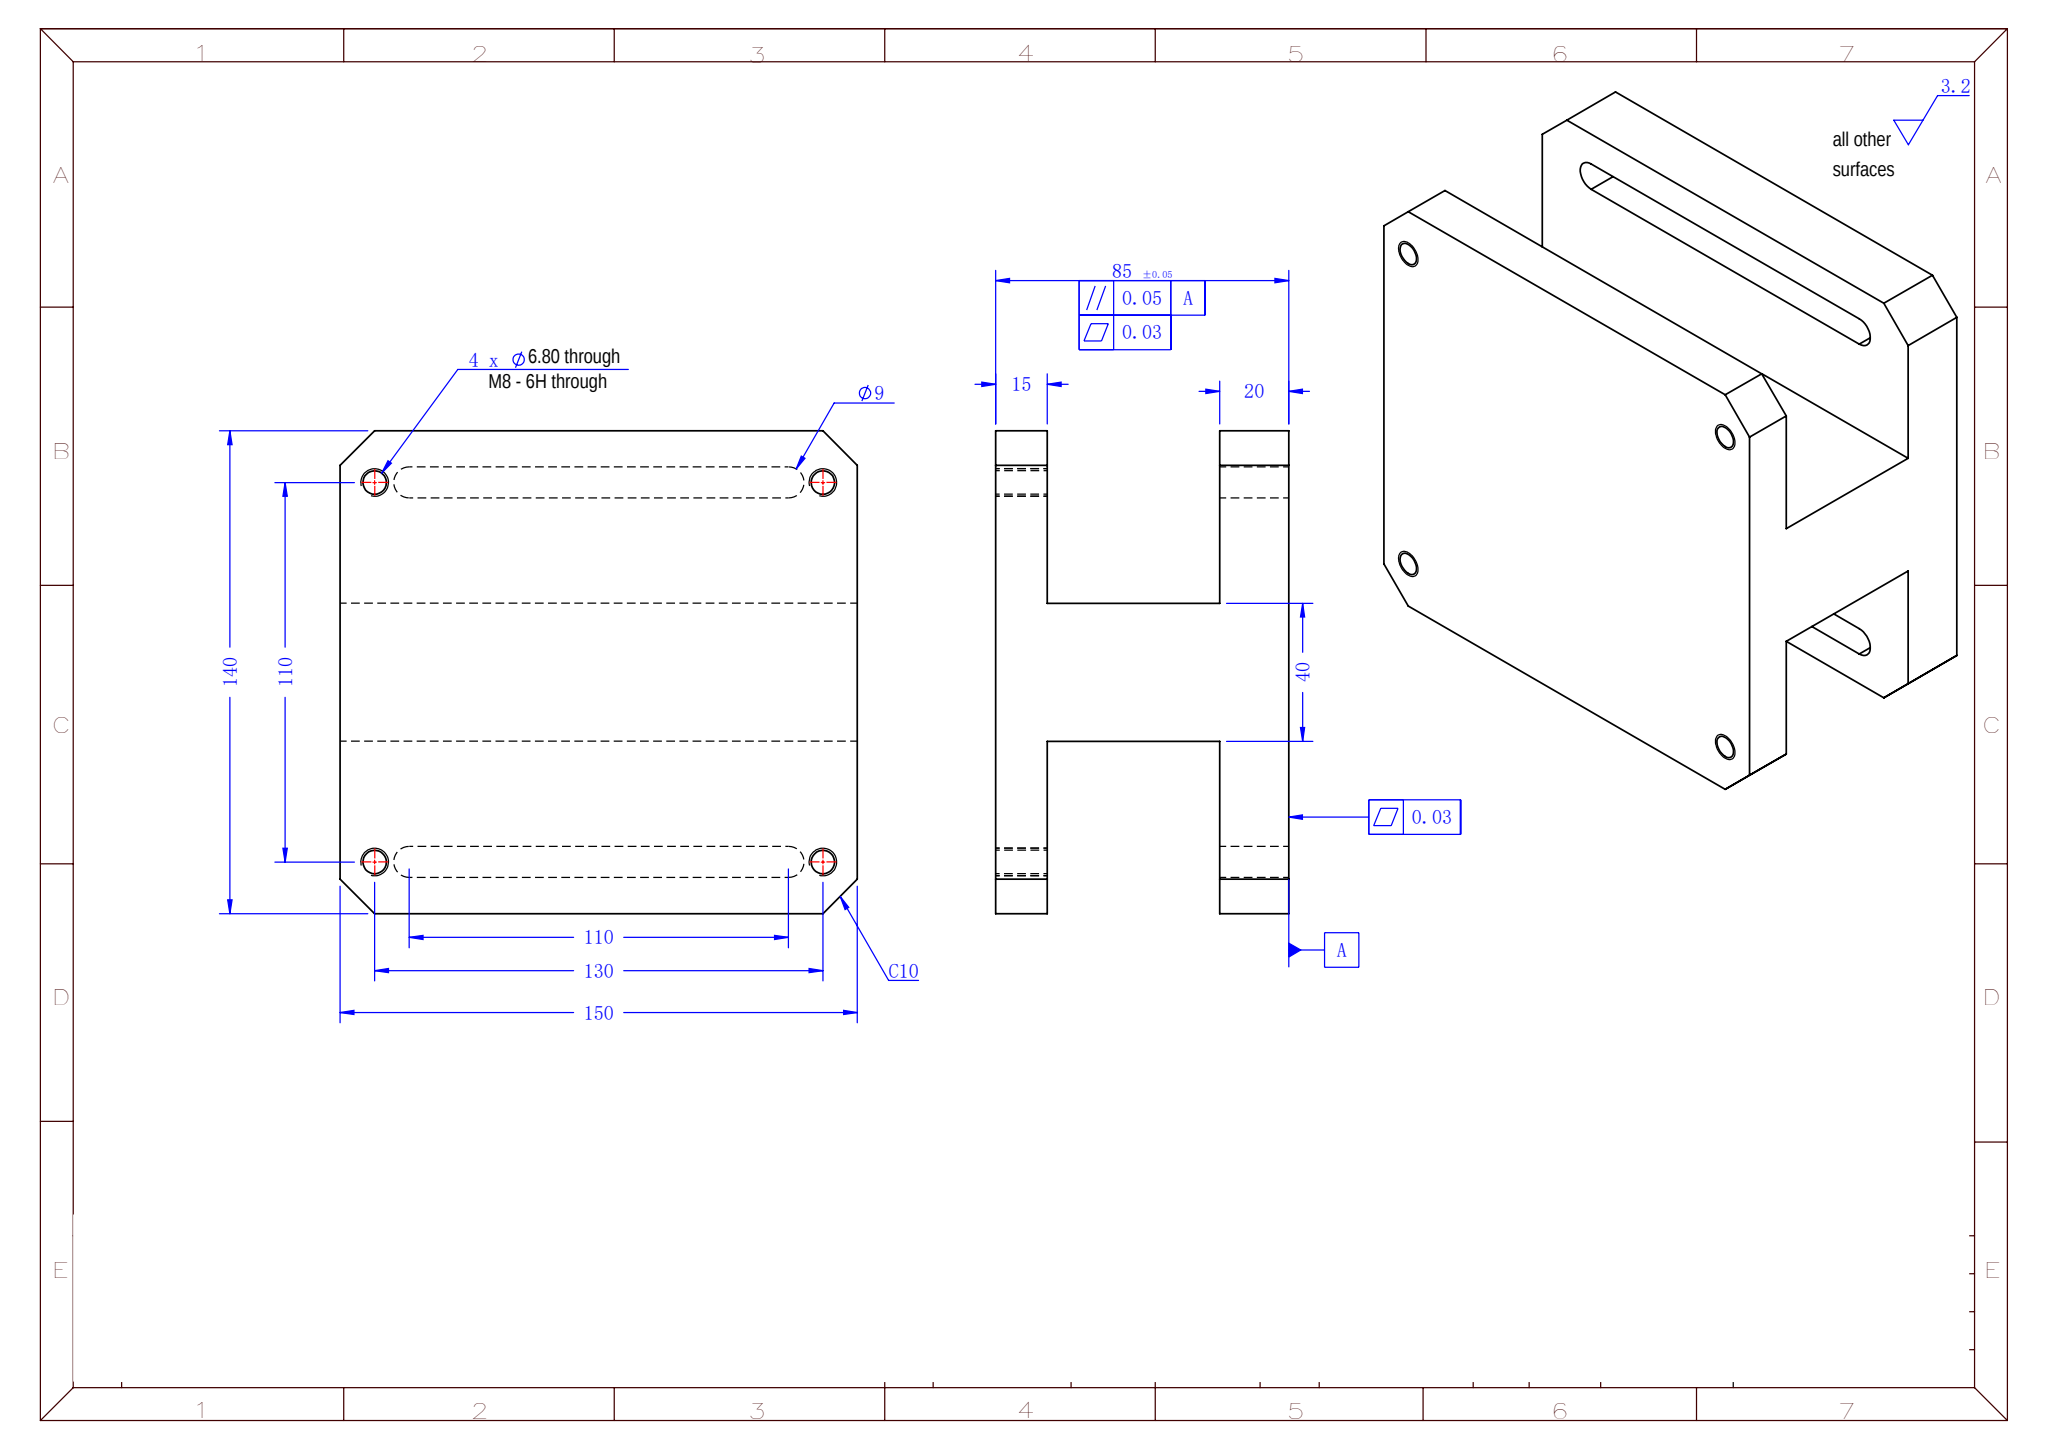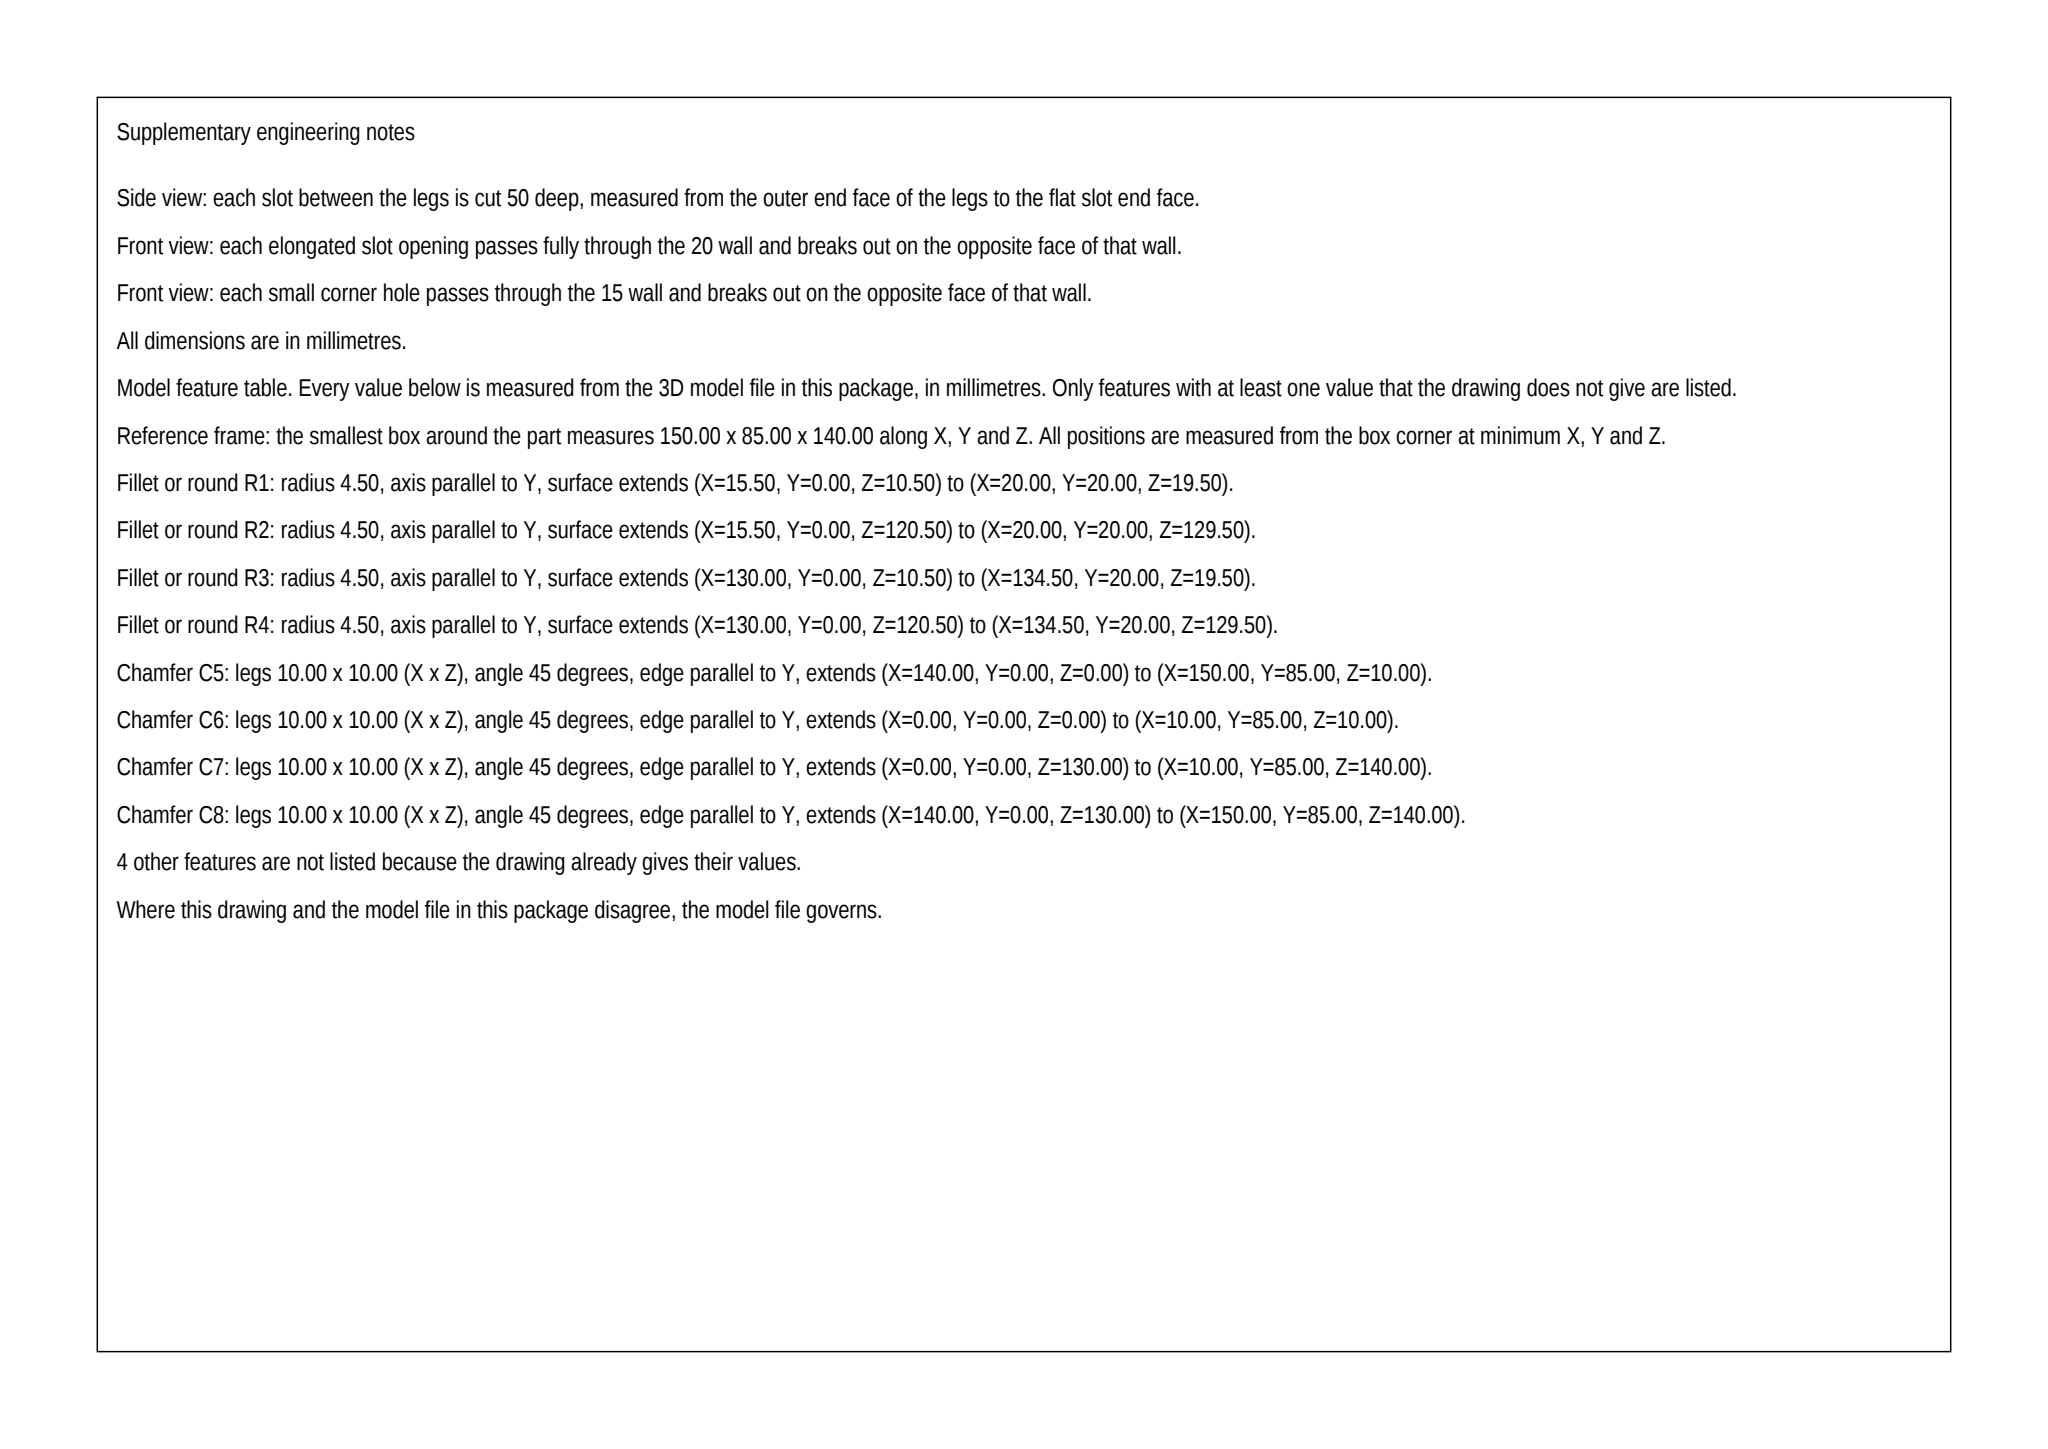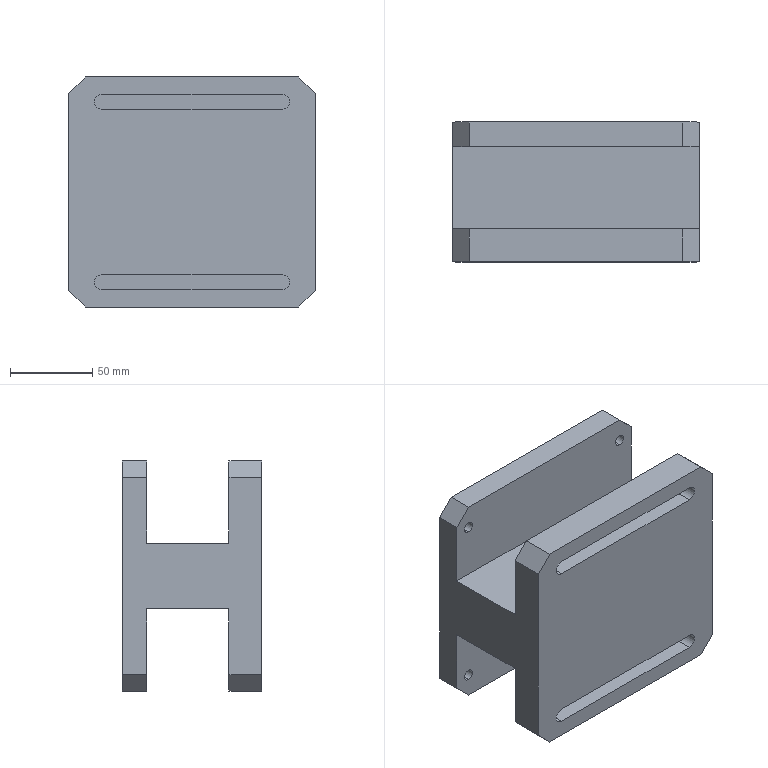Part | SolidWorks | mm | 1 solid | 38 faces | box 150 x 85 x 140 mm | volume 983676 mm3 | plane 26 | cylinder 12 | commonest cylinder face diameters 6.8 x8 9 x4
build123d program:
from build123d import *

# Parameters (mm, degrees)
SKETCH1_W             = 150
SKETCH1_H             = 85
BOSS_EXTRUDE1_DEPTH   = 70
SKETCH2_W             = 50
SKETCH2_H             = 50
CUT_EXTRUDE1_DEPTH    = 171.898
M8_TAPPED_HOLE1_D     = 6.8
M8_TAPPED_HOLE1_DEPTH = 15
CUT_EXTRUDE2_REACH    = 135.229
CHAMFER1_SIZE         = 10


with BuildPart() as part:
    # Sketch1 → Boss-Extrude1 (new, symmetric)
    with BuildSketch(Plane.XY):
        Rectangle(SKETCH1_W, SKETCH1_H)
    extrude(amount=BOSS_EXTRUDE1_DEPTH, both=True)

    # Sketch2 → Cut-Extrude1 (cut, through all)
    with BuildSketch(Plane(origin=(75, 0, 0), x_dir=(0, 0, -1), z_dir=(1, 0, 0))):
        with Locations((45, 2.5)):
            Rectangle(SKETCH2_W, SKETCH2_H)
    cut_extrude1 = extrude(amount=-CUT_EXTRUDE1_DEPTH, mode=Mode.SUBTRACT)

    # Mirror1: Cut-Extrude1 across plane
    add(cut_extrude1.mirror(Plane.XY), mode=Mode.SUBTRACT)

    # M8 Tapped Hole1
    with Locations(Plane(origin=(0, 42.5, 0), x_dir=(1, 0, 0), z_dir=(0, 1, 0))):
        with Locations((65, -55), (-65, -55), (65, 55), (-65, 55)):
            Hole(M8_TAPPED_HOLE1_D / 2, depth=M8_TAPPED_HOLE1_DEPTH)

    # Sketch9 → Cut-Extrude2 (cut, up to next)
    with BuildSketch(Plane.XZ.offset(42.5), mode=Mode.PRIVATE) as cut_extrude2_sk1:
        with BuildLine():
            Line((-55, 59.5), (55, 59.5))
            ThreePointArc((55, 59.5), (59.5, 55), (55, 50.5))
            Line((55, 50.5), (-55, 50.5))
            ThreePointArc((-55, 50.5), (-59.5, 55), (-55, 59.5))
        make_face()
    cut_extrude2_tool1 = extrude(cut_extrude2_sk1.sketch, amount=-CUT_EXTRUDE2_REACH, mode=Mode.PRIVATE) & part.part
    # Sketch9 → Cut-Extrude2 (cut, up to next)
    with BuildSketch(Plane.XZ.offset(42.5), mode=Mode.PRIVATE) as cut_extrude2_sk2:
        with BuildLine():
            Line((-55, -50.5), (55, -50.5))
            ThreePointArc((55, -50.5), (59.5, -55), (55, -59.5))
            Line((55, -59.5), (-55, -59.5))
            ThreePointArc((-55, -59.5), (-59.5, -55), (-55, -50.5))
        make_face()
    cut_extrude2_tool2 = extrude(cut_extrude2_sk2.sketch, amount=-CUT_EXTRUDE2_REACH, mode=Mode.PRIVATE) & part.part
    add(cut_extrude2_tool1.solids().sort_by_distance((0, -42.5, 55))[0], mode=Mode.SUBTRACT)
    add(cut_extrude2_tool2.solids().sort_by_distance((0, -42.5, -55))[0], mode=Mode.SUBTRACT)

    # Chamfer1
    chamfer1_edges = [part.edges().sort_by_distance(p)[0] for p in [
        (-75, 35, 70),
        (75, 35, -70),
        (-75, -32.5, -70),
        (75, 35, 70),
        (-75, -32.5, 70),
        (75, -32.5, 70),
        (-75, 35, -70),
        (75, -32.5, -70),
    ]]
    chamfer(chamfer1_edges, length=CHAMFER1_SIZE)


solid = part.part